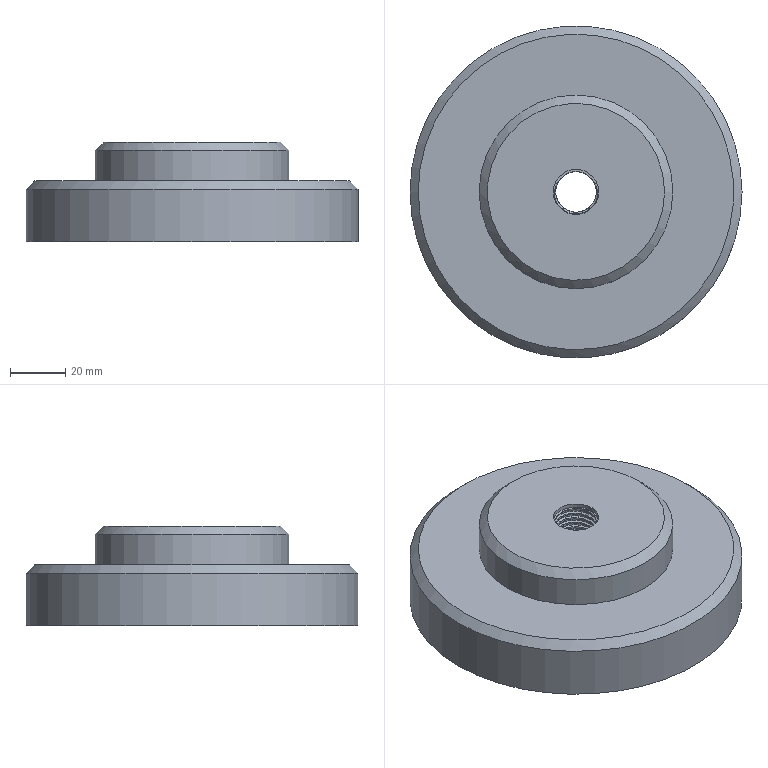Component | NX | Root-owned geometry | 1 solid | 16 faces | volume 225942 mm3 | cylinder 6 | plane 5 | spline 2 | cone 2 | torus 1 | commonest cylinder face diameters 120 x1 70 x1 90 x1 14.7 x1 16 x1 16.4 x1